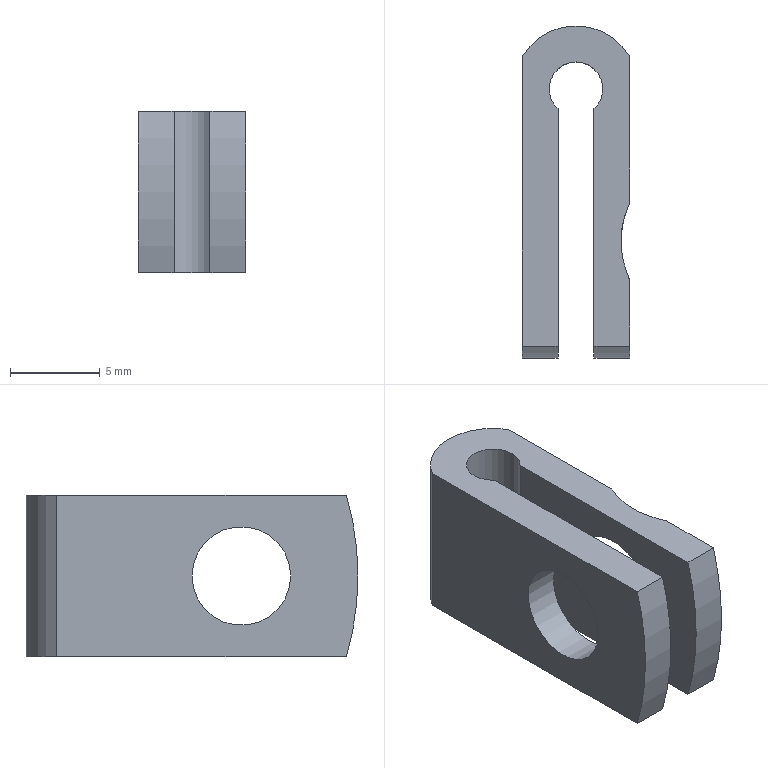Component | NX | 3_GAUGE_BASE | 1 solid | 13 faces | volume 506 mm3 | plane 7 | cylinder 5 | cone 1 | commonest cylinder face diameters 32 x2 7 x1 3 x1 5.5 x1